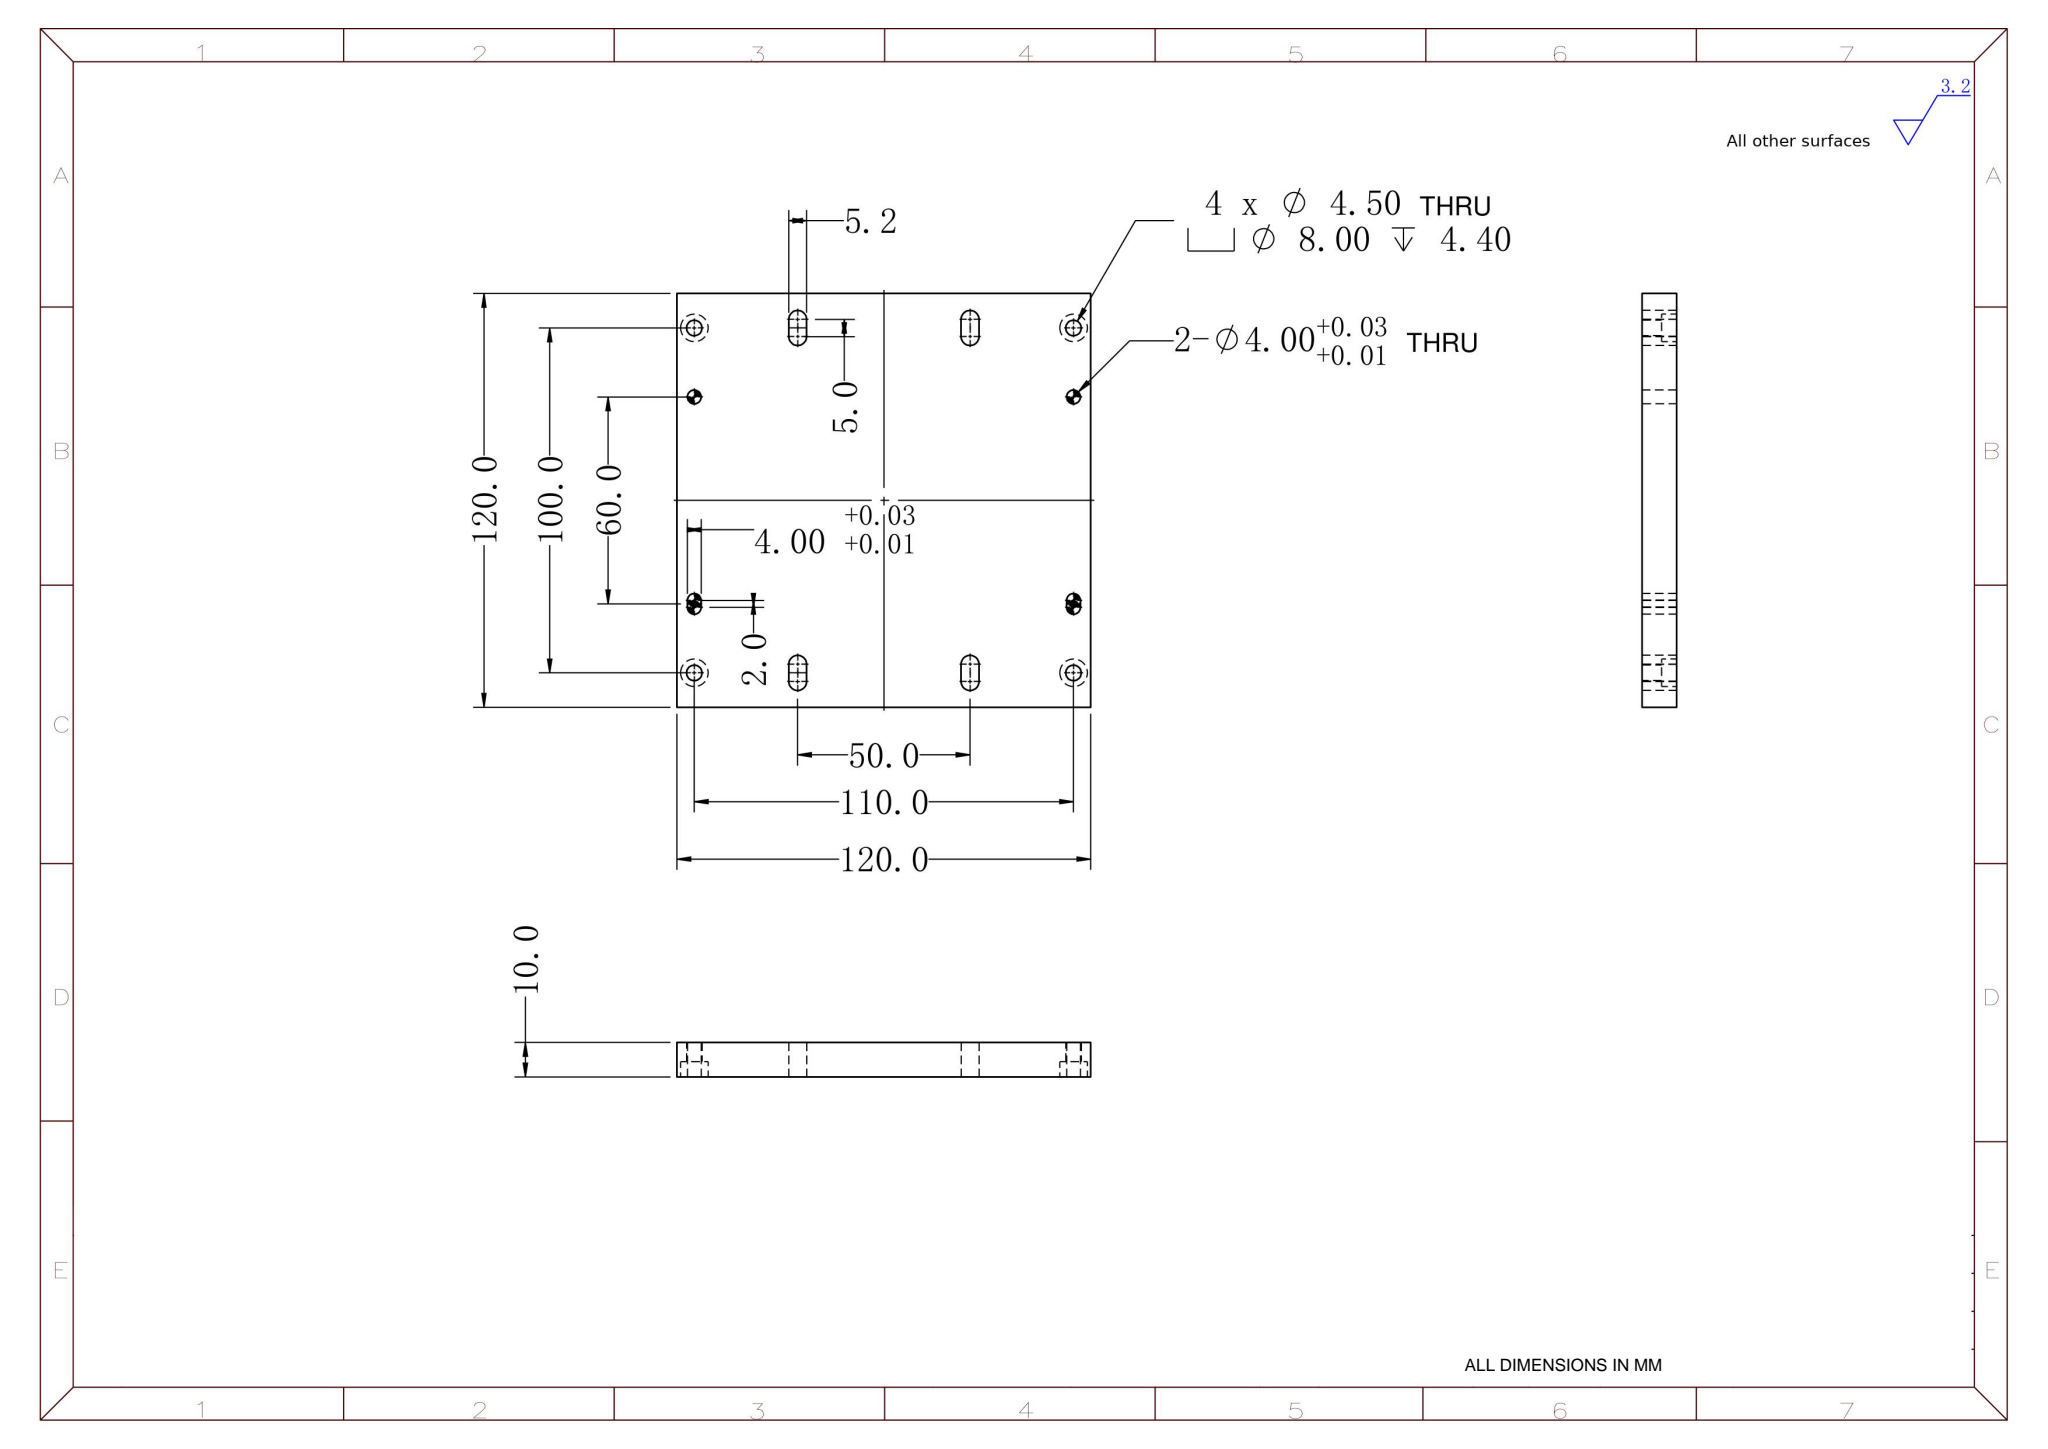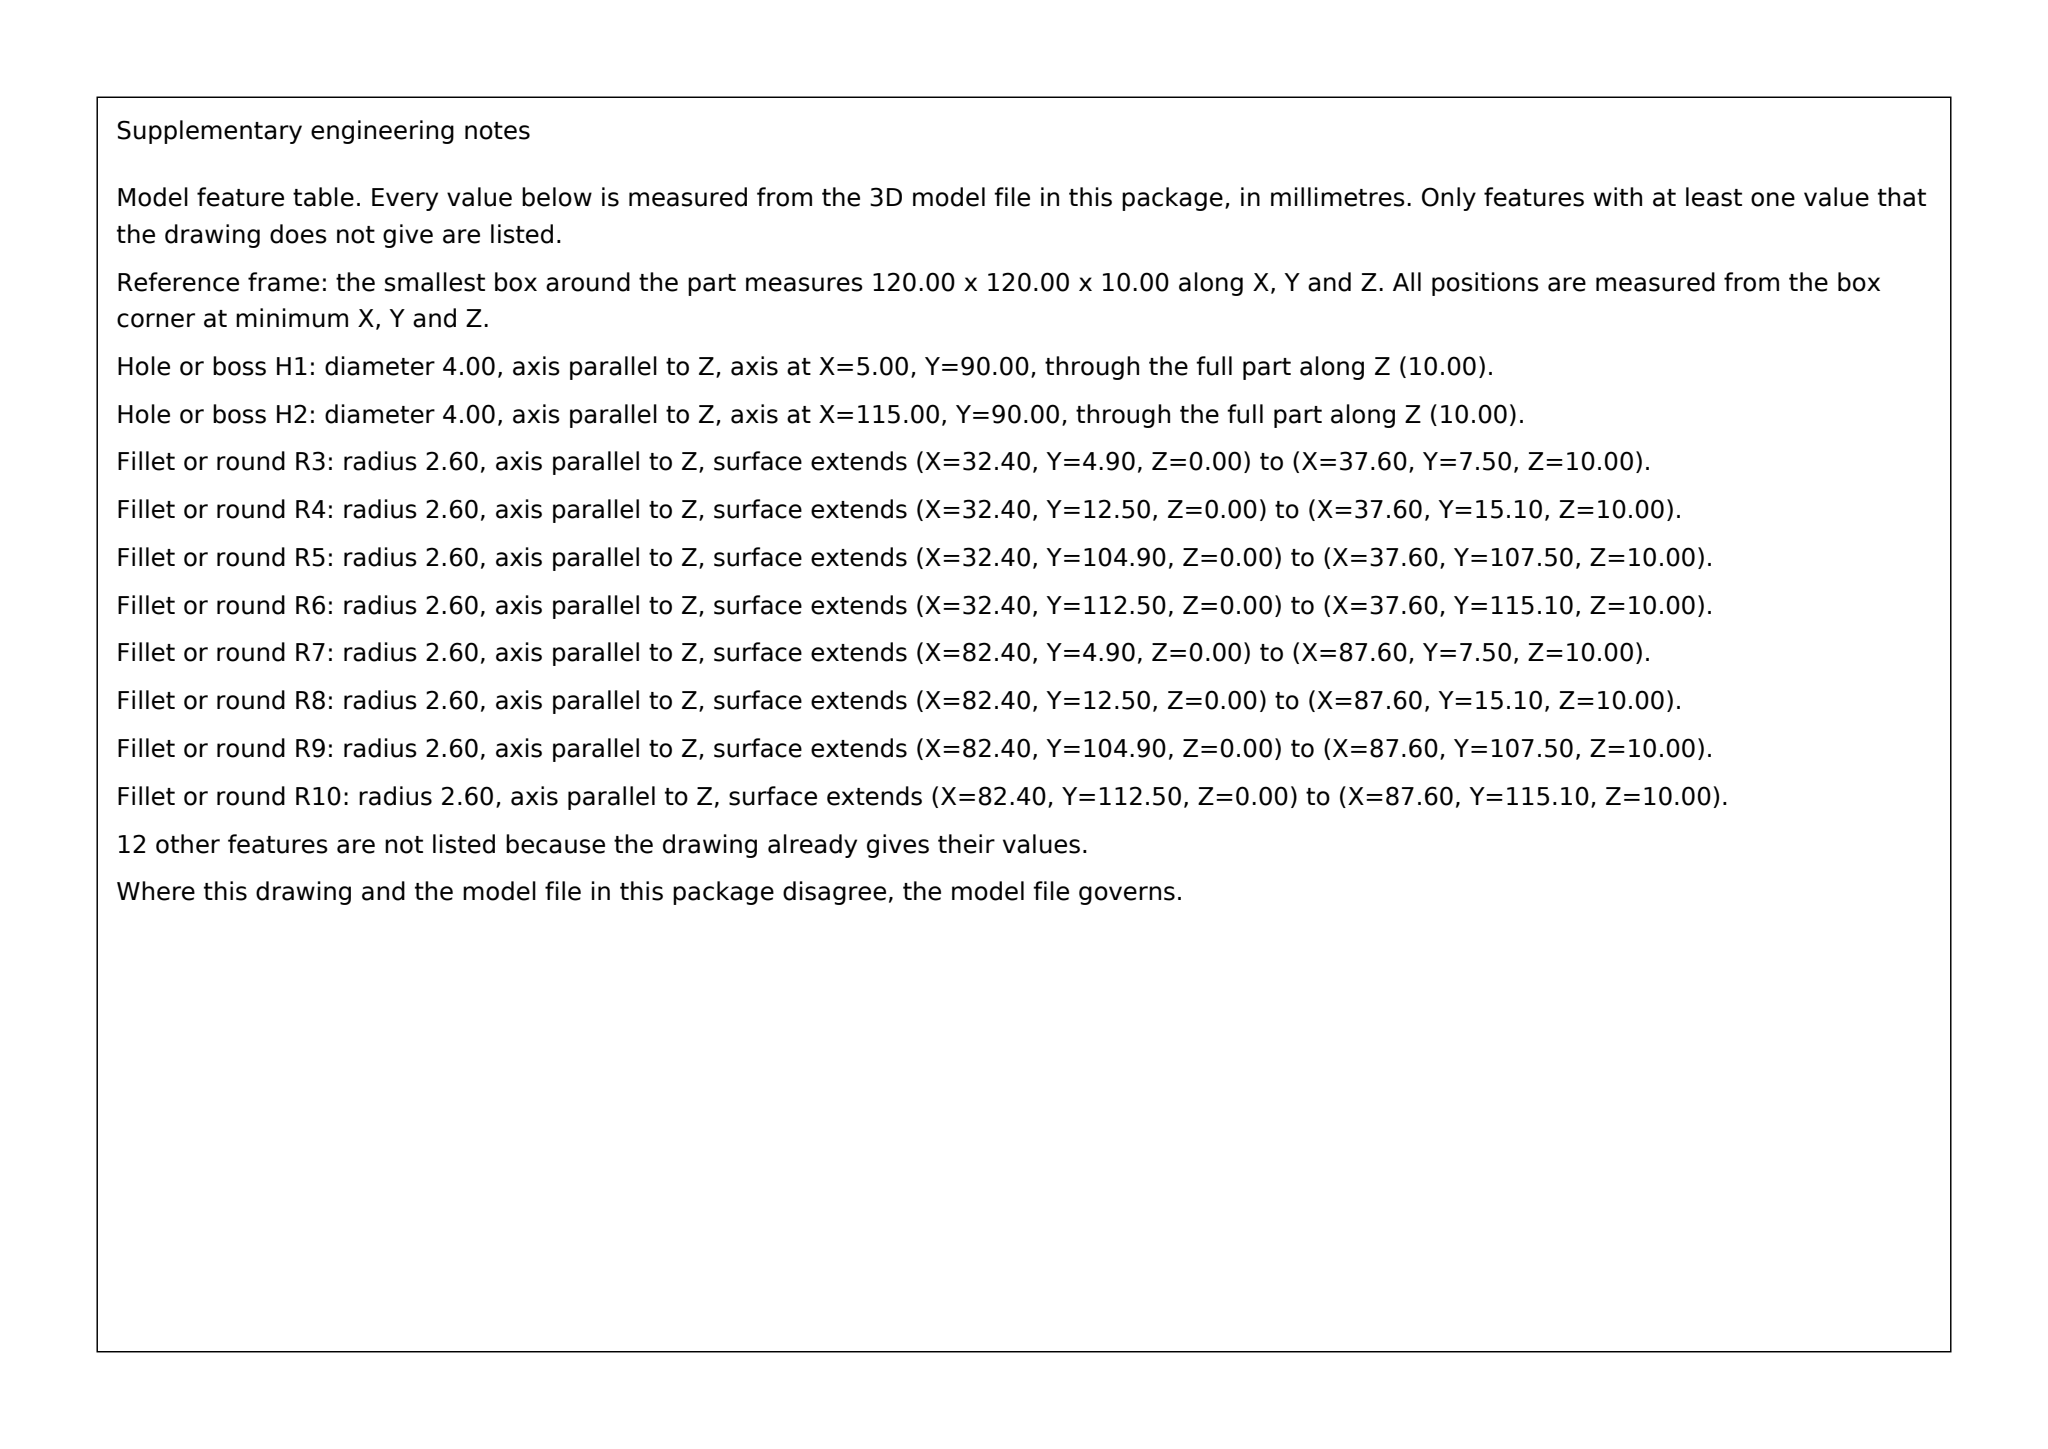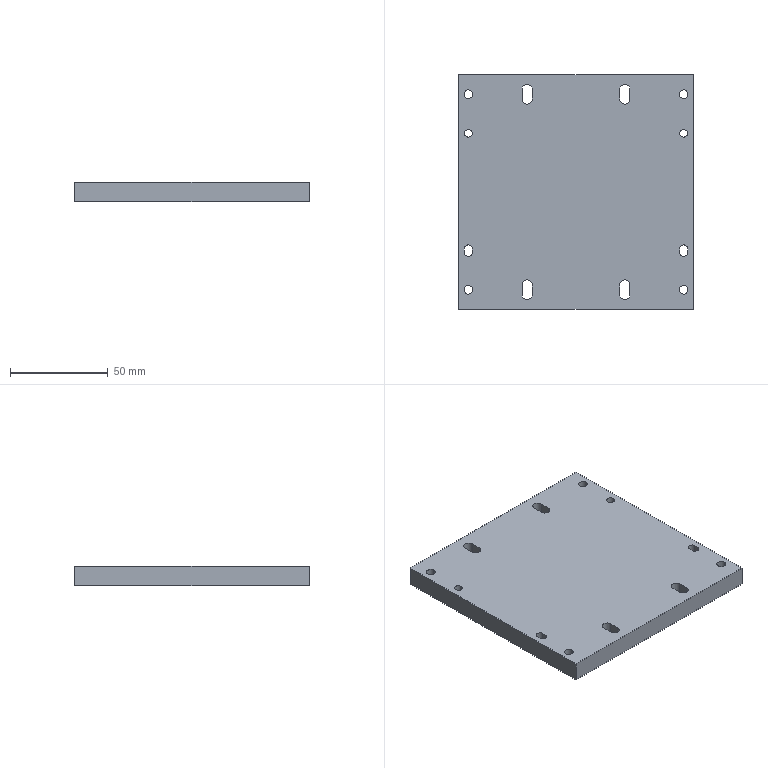Part | SolidWorks | mm | 1 solid | 54 faces | box 120 x 120 x 10 mm | volume 140207 mm3 | cylinder 32 | plane 22 | commonest cylinder face diameters 8 x8 4.5 x8 4 x8 5.2 x8
build123d program:
from build123d import *

# Parameters (mm, degrees)
SKETCH1_W                                       = 120
SKETCH1_H                                       = 120
SKETCH1_R                                       = 2
BOSS_EXTRUDE1_DEPTH                             = 5
M4_HEX_SOCKET_HEAD_CAP_SCREW_CBORE2_D           = 4.5
M4_HEX_SOCKET_HEAD_CAP_SCREW_CBORE2_CBORE_D     = 8
M4_HEX_SOCKET_HEAD_CAP_SCREW_CBORE2_CBORE_DEPTH = 4.4


with BuildPart() as part:
    # Sketch1 → Boss-Extrude1 (new, symmetric)
    with BuildSketch(Plane.XY):
        Rectangle(SKETCH1_W, SKETCH1_H)
        with Locations((55, 30)):
            Circle(SKETCH1_R, mode=Mode.SUBTRACT)
        with Locations(Location((-55, 30, 0), (0, 0, 180))):
            Circle(SKETCH1_R, mode=Mode.SUBTRACT)
        with BuildLine():
            Line((57, -29), (57, -31))
            ThreePointArc((57, -31), (55, -33), (53, -31))
            Line((53, -31), (53, -29))
            ThreePointArc((53, -29), (55, -27), (57, -29))
        make_face(mode=Mode.SUBTRACT)
        with BuildLine():
            Line((-57, -29), (-57, -31))
            ThreePointArc((-57, -31), (-55, -33), (-53, -31))
            Line((-53, -31), (-53, -29))
            ThreePointArc((-53, -29), (-55, -27), (-57, -29))
        make_face(mode=Mode.SUBTRACT)
        with BuildLine():
            Line((27.6, -47.5), (27.6, -52.5))
            ThreePointArc((27.6, -52.5), (25, -55.1), (22.4, -52.5))
            Line((22.4, -52.5), (22.4, -47.5))
            ThreePointArc((22.4, -47.5), (25, -44.9), (27.6, -47.5))
        make_face(mode=Mode.SUBTRACT)
        with BuildLine():
            Line((27.6, 47.5), (27.6, 52.5))
            ThreePointArc((27.6, 52.5), (25, 55.1), (22.4, 52.5))
            Line((22.4, 52.5), (22.4, 47.5))
            ThreePointArc((22.4, 47.5), (25, 44.9), (27.6, 47.5))
        make_face(mode=Mode.SUBTRACT)
        with BuildLine():
            Line((-27.6, -47.5), (-27.6, -52.5))
            ThreePointArc((-27.6, -52.5), (-25, -55.1), (-22.4, -52.5))
            Line((-22.4, -52.5), (-22.4, -47.5))
            ThreePointArc((-22.4, -47.5), (-25, -44.9), (-27.6, -47.5))
        make_face(mode=Mode.SUBTRACT)
        with BuildLine():
            Line((-27.6, 47.5), (-27.6, 52.5))
            ThreePointArc((-27.6, 52.5), (-25, 55.1), (-22.4, 52.5))
            Line((-22.4, 52.5), (-22.4, 47.5))
            ThreePointArc((-22.4, 47.5), (-25, 44.9), (-27.6, 47.5))
        make_face(mode=Mode.SUBTRACT)
    extrude(amount=BOSS_EXTRUDE1_DEPTH, both=True)

    # M4 Hex Socket Head Cap Screw CBORE2 (through all)
    with Locations(Plane(origin=(0, 0, -5), x_dir=(-1, 0, 0), z_dir=(0, 0, -1))):
        with Locations((55, -50), (55, 50), (-55, 50), (-55, -50)):
            CounterBoreHole(M4_HEX_SOCKET_HEAD_CAP_SCREW_CBORE2_D / 2, M4_HEX_SOCKET_HEAD_CAP_SCREW_CBORE2_CBORE_D / 2, M4_HEX_SOCKET_HEAD_CAP_SCREW_CBORE2_CBORE_DEPTH)


solid = part.part